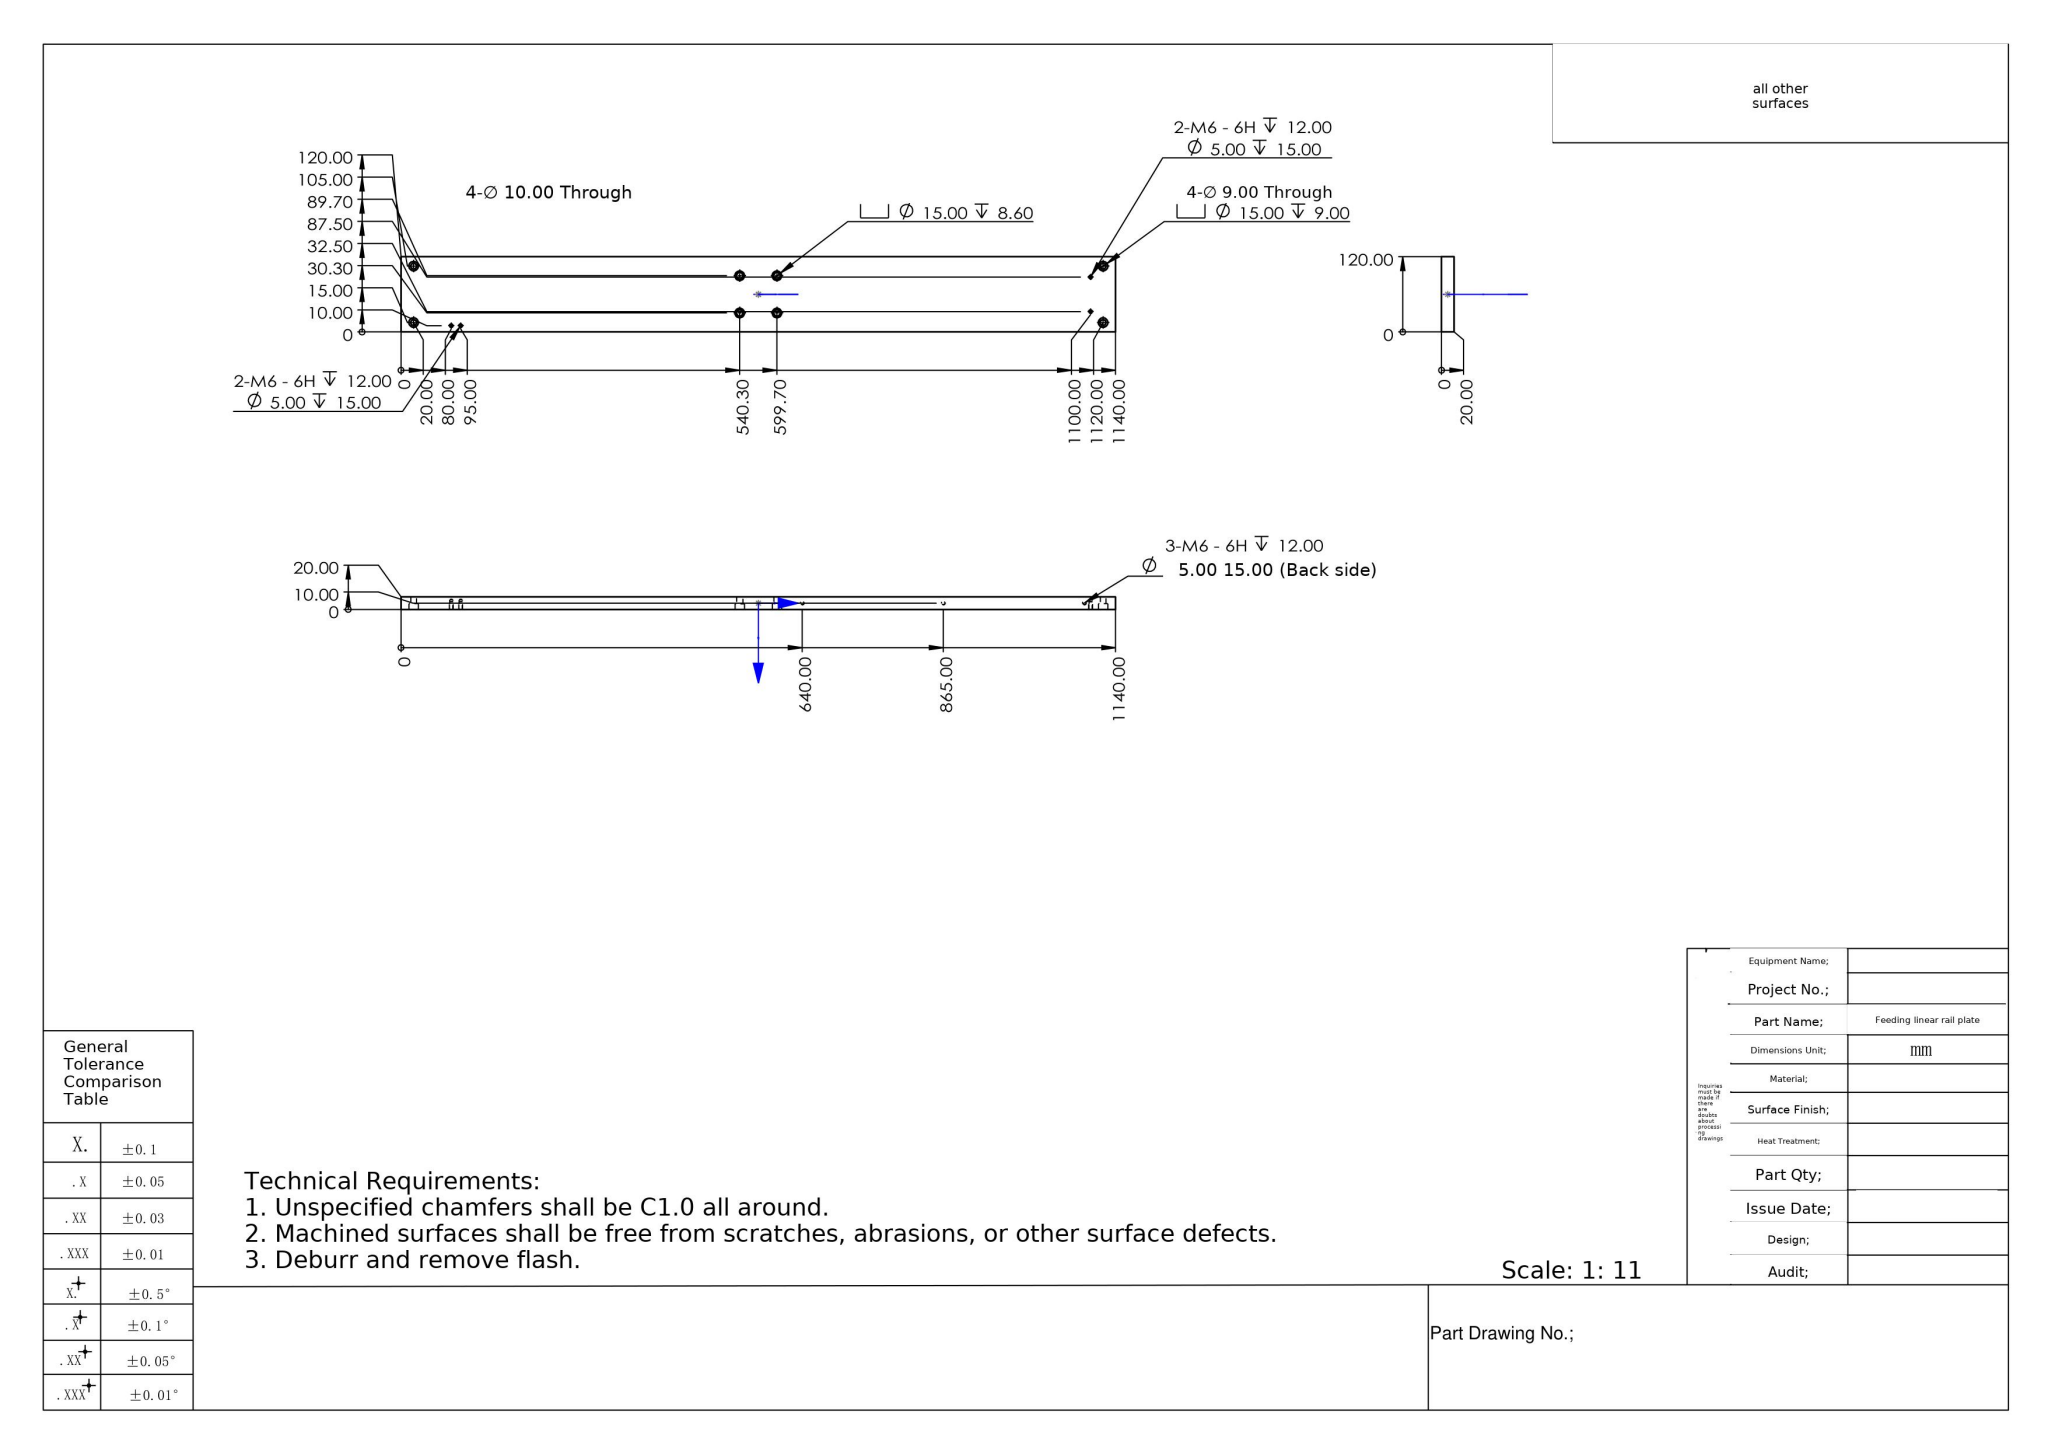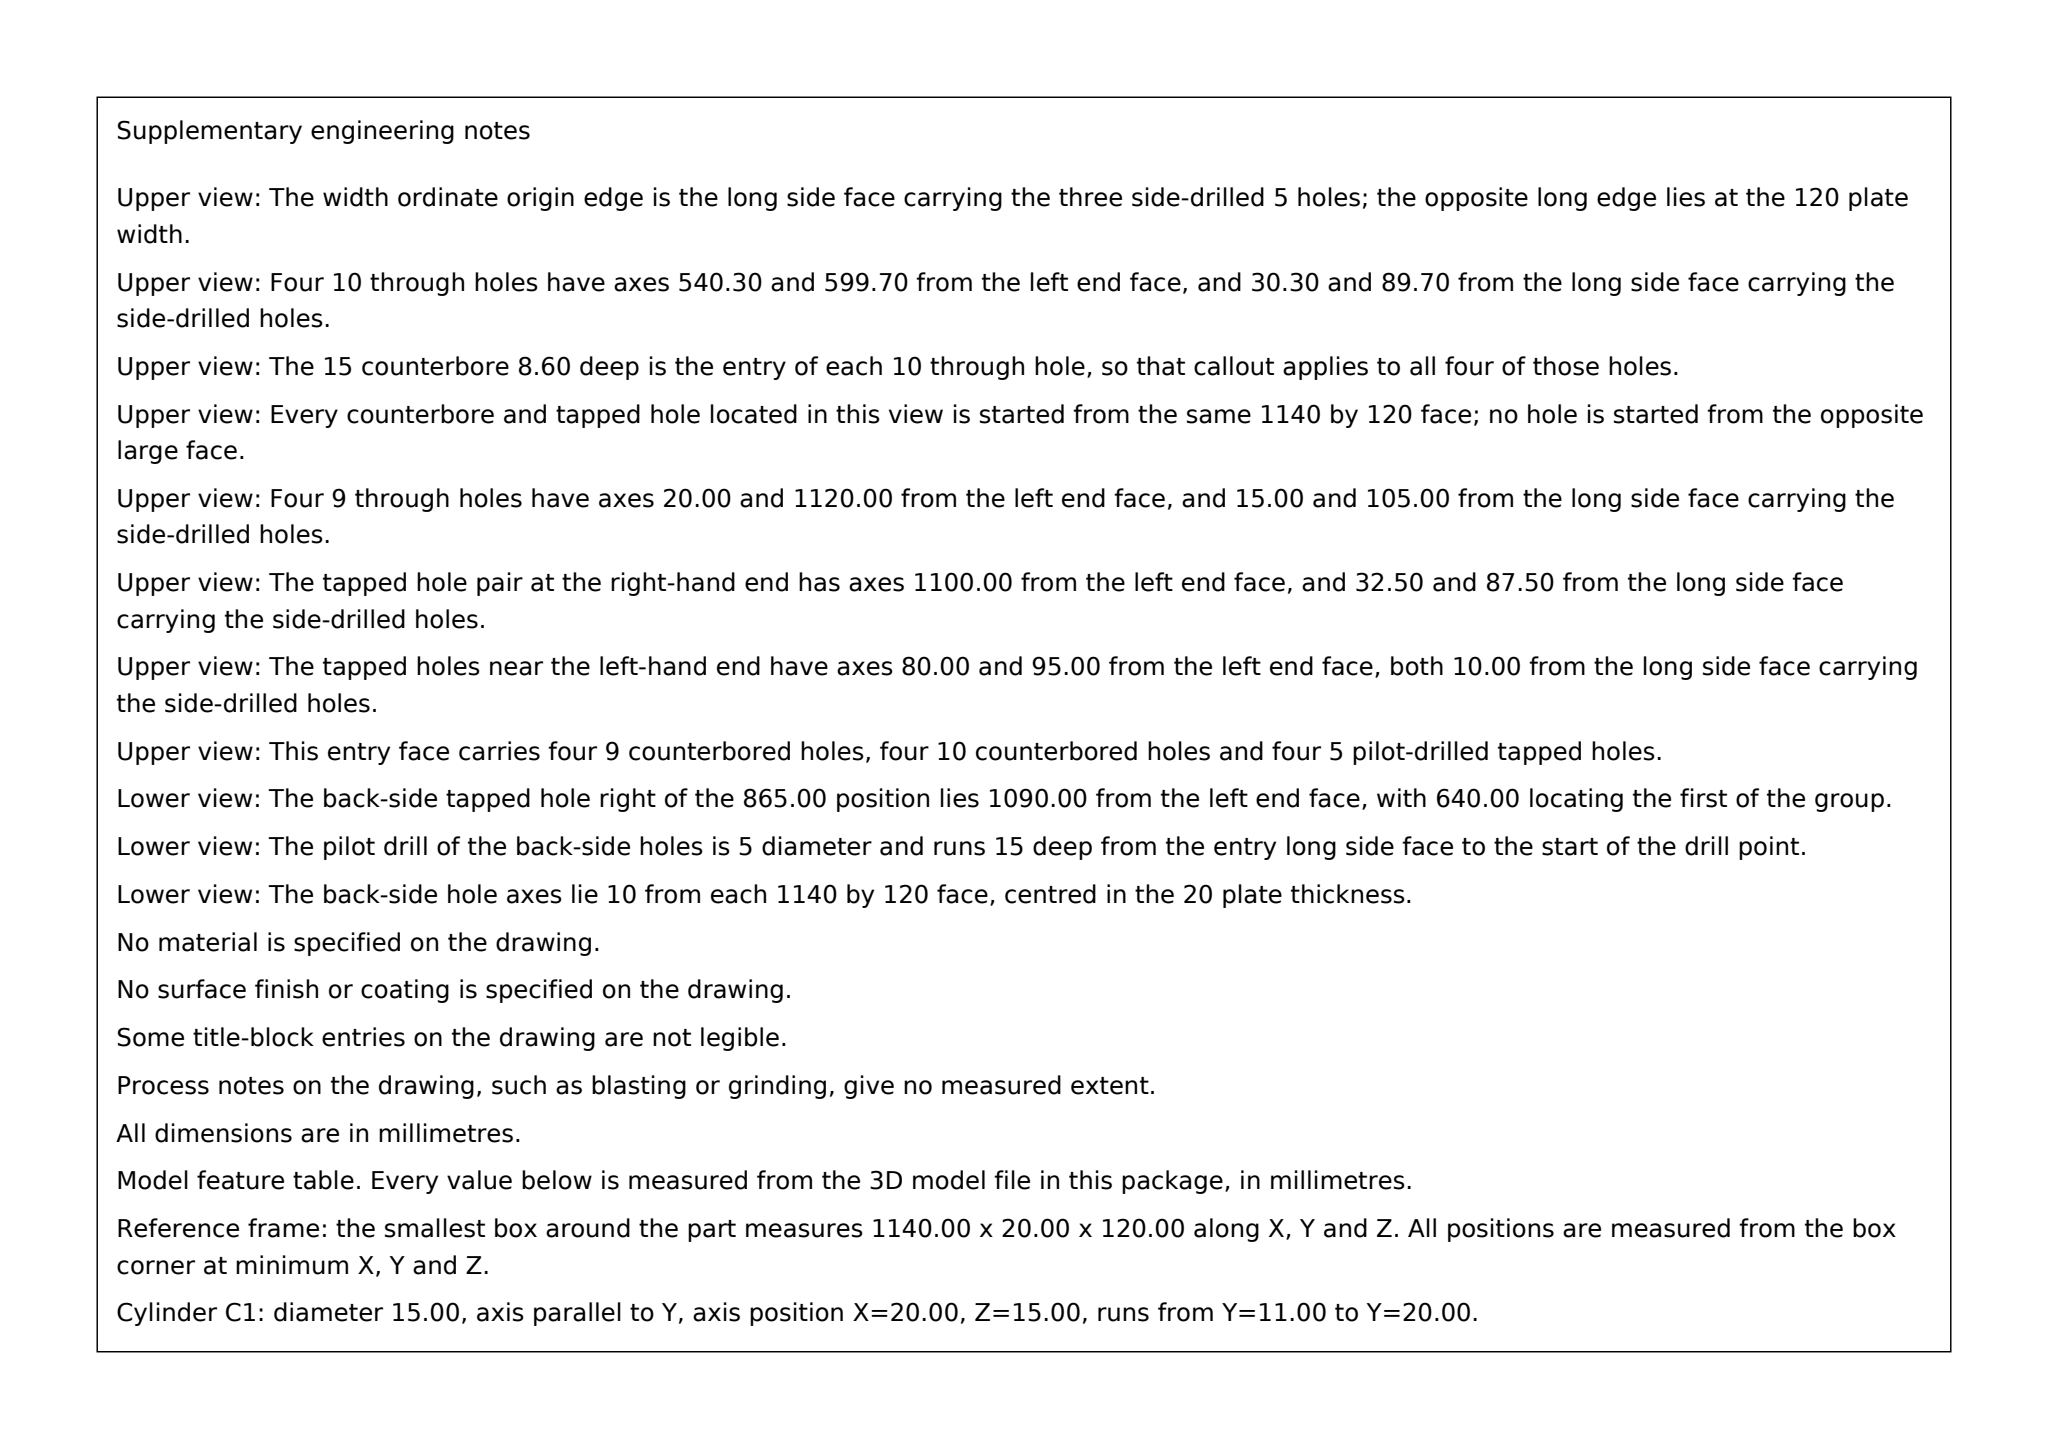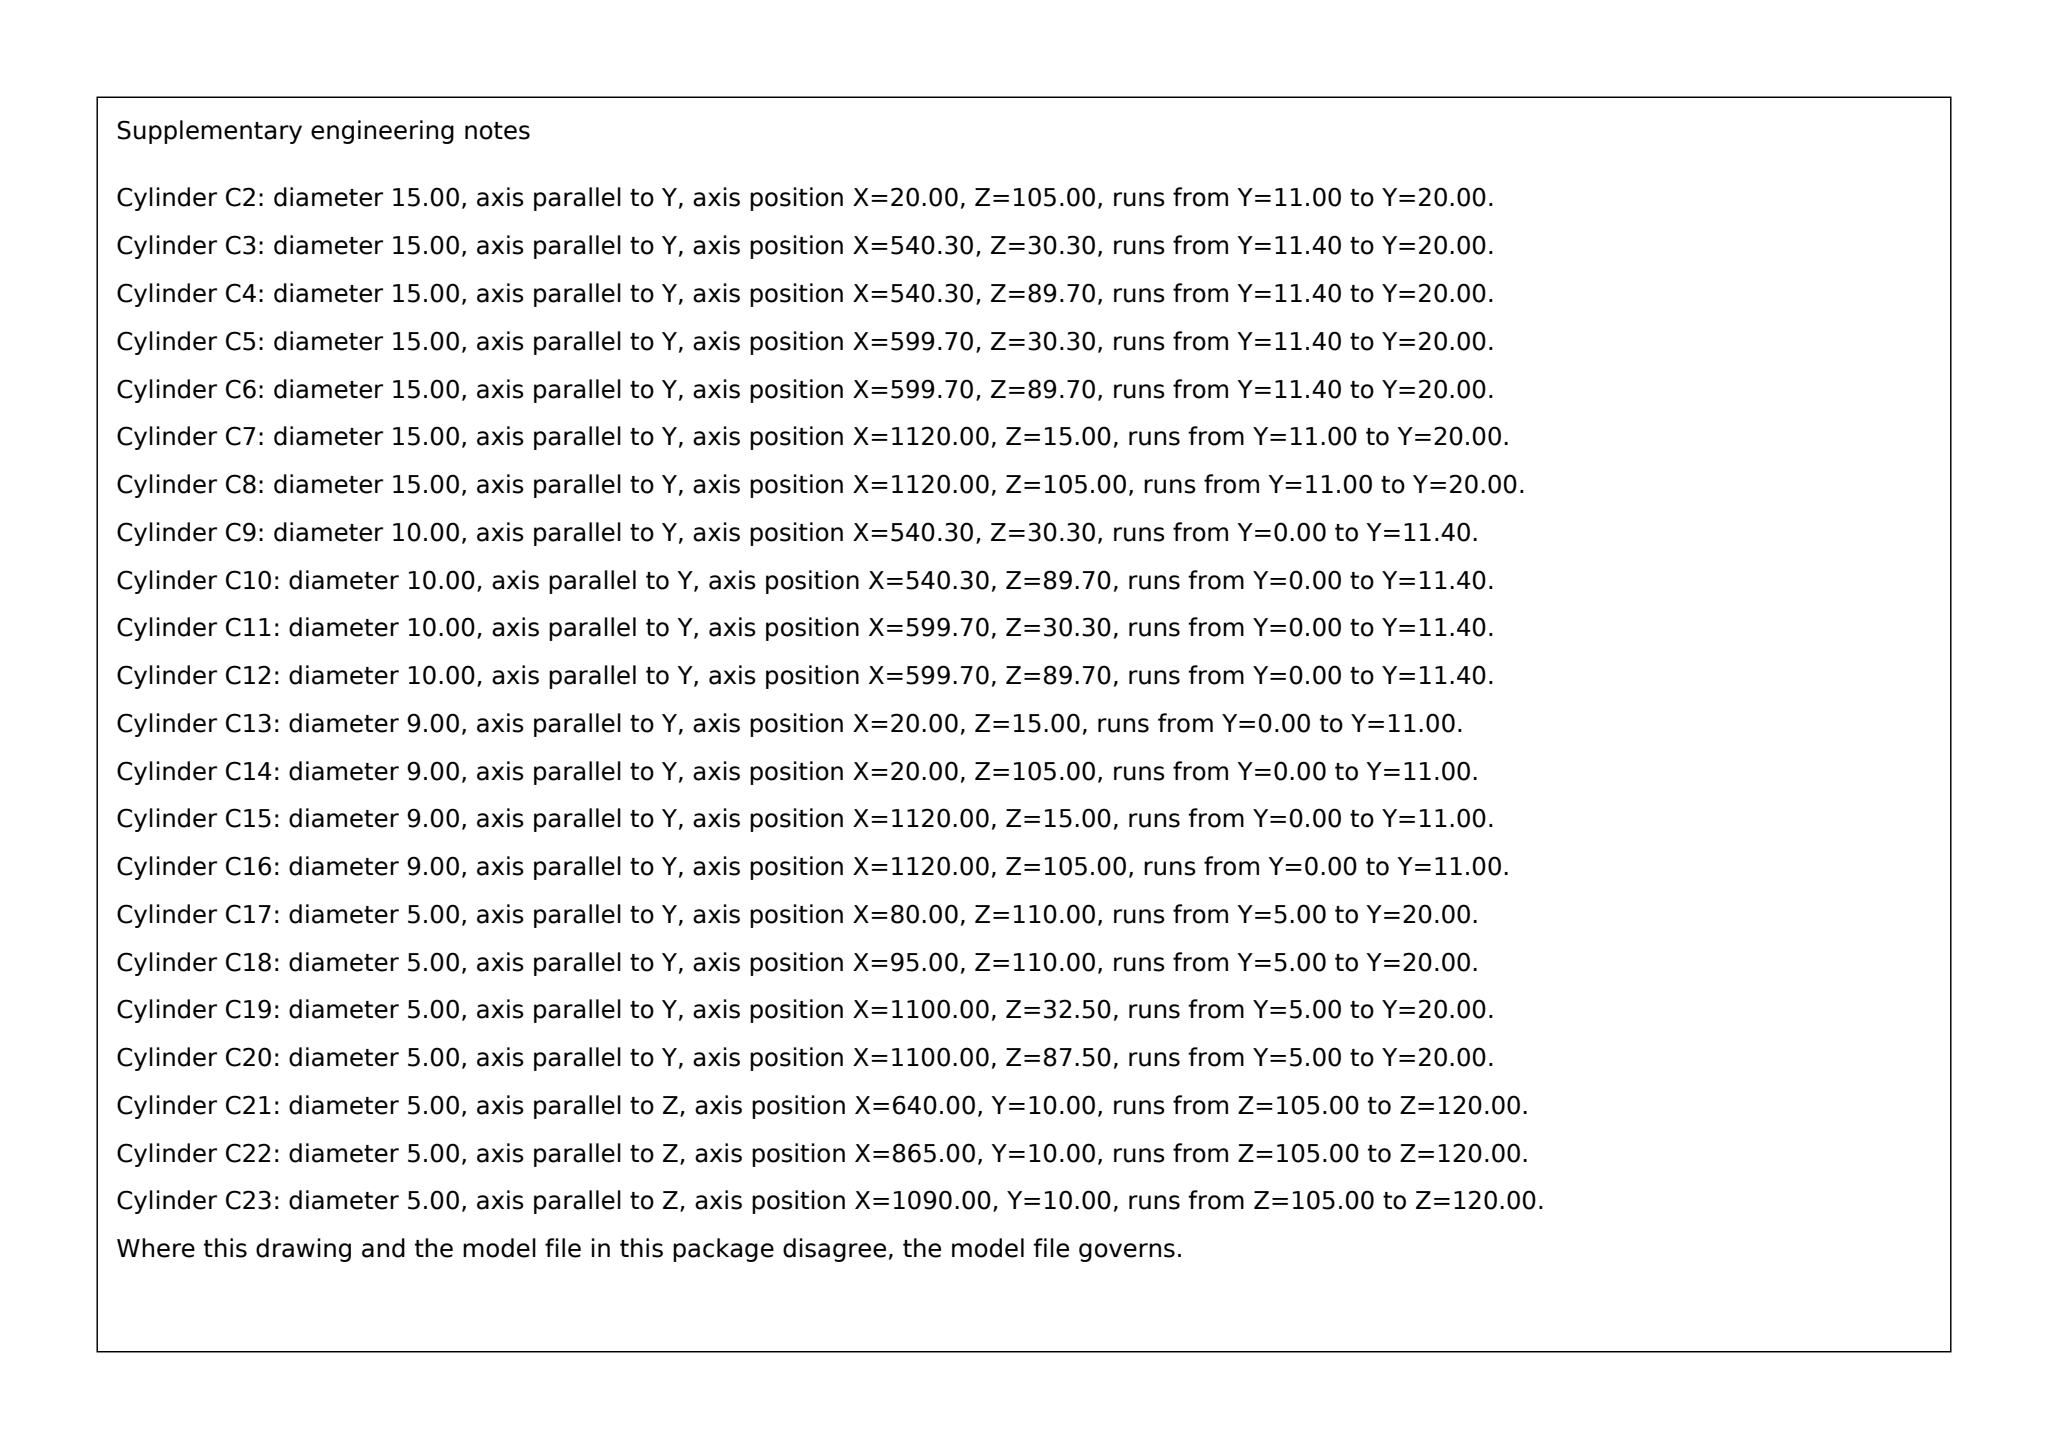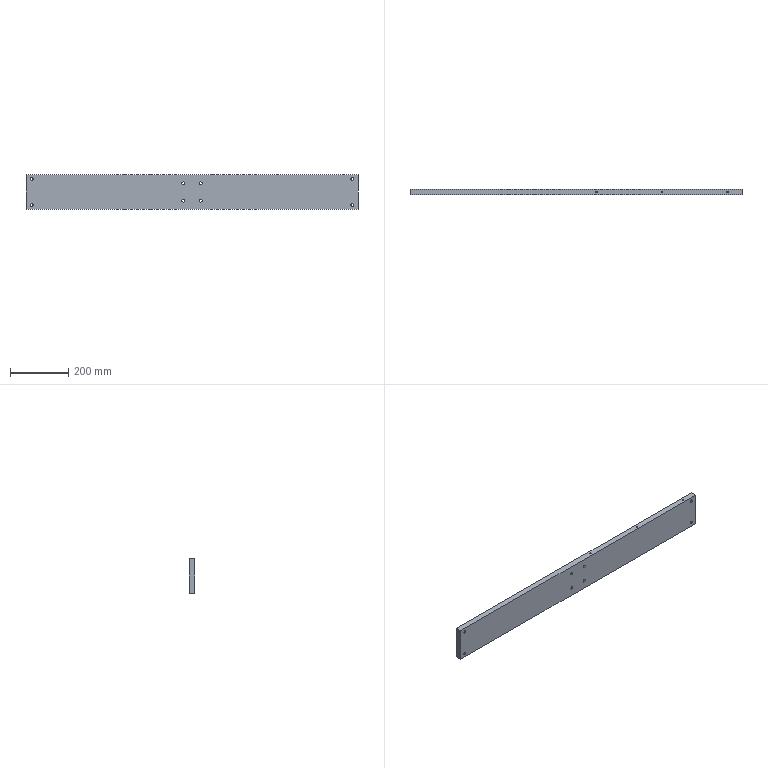Part | SolidWorks | mm | 1 solid | 74 faces | box 1140 x 20 x 120 mm | volume 2715048 mm3 | cylinder 46 | cone 14 | plane 14 | commonest cylinder face diameters 15 x16 5 x14 10 x8 9 x8
Drawing notes:
4X Ø9 C'BORE Ø15 DP 9.00 (AT X=20 & X=1120, Z=15 & Z=105) IS MACHINED FROM THE Y=20.00 FACE (C'BORE FLAT AT Y=11.00 FROM Y=0 DATUM FACE). | from the solid: cylinders [15.0,'y',[20.0,null,15.0],9.0] and [15.0,'y',[1120.0,null,105.0],9.0] with axis_planes ['y',11.0,4] = 20.00-9.00, so c'bores open at Y=20
3X M6-6H DP 12 / DRILL Ø5.00 DP 15.00, AXIS PARALLEL TO Z, AT X=640.00, 865.00, 1090.00, Y=10.00 FROM MIN CORNER. | from the solid: cylinders [5.0,'z',[640.0,10.0,null],15.0], [5.0,'z',[865.0,10.0,null],15.0], [5.0,'z',[1090.0,10.0,null],15.0]
4X M6-6H TAPPED HOLE DP 12 / DRILL Ø5.00 DP 15.00, AXIS PARALLEL TO Y, ENTERED FROM THE Y=20.00 FACE (DRILL BOTTOMS AT Y=5.00), AT X=80.00 & X=95.00 (Z=110.00) AND X=1100.00 (Z=32.50 & Z=87.50), ALL FROM MIN CORNER OF 1140 x 20 x 120 BODY | from the solid: cylinders: 4X dia 5.0 axis y at (80,-,110),(95,-,110),(1100,-,32.5),(1100,-,87.5) from y=5.0 to y=20.0; axis_planes y=20.0 full face
4X Ø10 THRU; CBORE Ø15 DP 8.6 FR Y=20 FACE (BACK SIDE) | from the solid: Ø10 y-holes y0→11.4 at X540.3/599.7, Z30.3/89.7; Ø15 y-bores y11.4→20 same axes (8.6 deep)
4X M6-6H DP 12; DRILL Ø5 DP 15; AXIS PARALLEL Y; FR Y=20 FACE | from the solid: Ø5 y-holes y5→20 (15 deep) at (1100,32.5),(1100,87.5),(80,110),(95,110)
M6 PARALLEL Y LOC: X80 & X95 @ Z110; X1100 @ Z32.5 & Z87.5 | from the solid: Ø5 y-axis hole positions [80,110],[95,110],[1100,32.5],[1100,87.5]
M6-6H DP 12; DRILL Ø5 DP 15; AXIS PARALLEL Z; X=1090, Y=10; FR Z=120 | from the solid: Ø5 z-hole at (1090,10), z105→120, 15 deep from Z=120 face
X=1090: 1 M6 HOLE ONLY - DELETE DUPLICATE CALLOUT | from the solid: only one Ø5 z-cylinder at (1090,10,z105-120) in model
3X M6-6H DP 12; Ø5 DP 15 (BACK) AT X=640, 865, 1090; Y=10 | from the solid: Ø5 z-holes at (640,10),(865,10),(1090,10), z105→120
X=1090 M6 AXIS PARALLEL Z, ENTERS Z=120 FACE, Y=10, 1 PLC | from the solid: z-axis Ø5 hole (1090,10) runs z105→120; entry at Z=120 plane
Ø5 DP 15 (BACK) APPLIES TO ALL 3 PARALLEL Z M6: X640/865/1090 | from the solid: three Ø5 z-holes each 15 deep from Z=120 face, Y=10
build123d program:
from build123d import *

# Parameters (mm, degrees)
SKETCH1_W                                            = 1140
SKETCH1_H                                            = 20
BOSS_EXTRUDE1_DEPTH                                  = 60
HOLE_SIZE_ACCORDING_TO_THE_TYPE_OF_HEX_S_D           = 9
HOLE_SIZE_ACCORDING_TO_THE_TYPE_OF_HEX_S_CBORE_D     = 15
HOLE_SIZE_ACCORDING_TO_THE_TYPE_OF_HEX_S_CBORE_DEPTH = 9
M6_TAPPED_HOLE1_D                                    = 5
M6_TAPPED_HOLE1_DEPTH                                = 15
M6_TAPPED_HOLE1_TIP                                  = 1.502
M8_HEX_SOCKET_HEAD_CAP_SCREW_CBORE1_D                = 10
M8_HEX_SOCKET_HEAD_CAP_SCREW_CBORE1_CBORE_D          = 15
M8_HEX_SOCKET_HEAD_CAP_SCREW_CBORE1_CBORE_DEPTH      = 8.6
M6_TAPPED_HOLE2_D                                    = 5
M6_TAPPED_HOLE2_DEPTH                                = 15
M6_TAPPED_HOLE2_TIP                                  = 1.502
M6_TAPPED_HOLE3_D                                    = 5
M6_TAPPED_HOLE3_DEPTH                                = 15
M6_TAPPED_HOLE3_TIP                                  = 1.502


with BuildPart() as part:
    # Sketch1 → Boss-Extrude1 (new, symmetric)
    with BuildSketch(Plane.XY):
        Rectangle(SKETCH1_W, SKETCH1_H)
    extrude(amount=BOSS_EXTRUDE1_DEPTH, both=True)

    # Hole Size according to the type of Hex S (through all)
    with Locations(Plane(origin=(0, 10, 0), x_dir=(1, 0, 0), z_dir=(0, 1, 0))):
        with Locations((-550, 45), (-550, -45), (550, 45), (550, -45)):
            CounterBoreHole(HOLE_SIZE_ACCORDING_TO_THE_TYPE_OF_HEX_S_D / 2, HOLE_SIZE_ACCORDING_TO_THE_TYPE_OF_HEX_S_CBORE_D / 2, HOLE_SIZE_ACCORDING_TO_THE_TYPE_OF_HEX_S_CBORE_DEPTH)

    # M6 Tapped Hole1
    with Locations(Plane.XY.offset(60)):
        with Locations((70, 0), (295, 0), (520, 0)):
            Hole(M6_TAPPED_HOLE1_D / 2, depth=M6_TAPPED_HOLE1_DEPTH)
            with Locations((0, 0, -(M6_TAPPED_HOLE1_DEPTH + M6_TAPPED_HOLE1_TIP / 2))):  # 118° drill point
                Cone(0, M6_TAPPED_HOLE1_D / 2, M6_TAPPED_HOLE1_TIP, mode=Mode.SUBTRACT)

    # M8 Hex Socket Head Cap Screw CBORE1 (through all)
    with Locations(Plane(origin=(0, 10, 0), x_dir=(1, 0, 0), z_dir=(0, 1, 0))):
        with Locations((29.698, 29.698), (29.698, -29.698), (-29.698, -29.698), (-29.698, 29.698)):
            CounterBoreHole(M8_HEX_SOCKET_HEAD_CAP_SCREW_CBORE1_D / 2, M8_HEX_SOCKET_HEAD_CAP_SCREW_CBORE1_CBORE_D / 2, M8_HEX_SOCKET_HEAD_CAP_SCREW_CBORE1_CBORE_DEPTH)

    # M6 Tapped Hole2
    with Locations(Plane(origin=(23.67, 10, 26.577), x_dir=(1, 0, 0), z_dir=(0, 1, 0))):
        with Locations((-513.67, -23.423), (-498.67, -23.423)):
            Hole(M6_TAPPED_HOLE2_D / 2, depth=M6_TAPPED_HOLE2_DEPTH)
            with Locations((0, 0, -(M6_TAPPED_HOLE2_DEPTH + M6_TAPPED_HOLE2_TIP / 2))):  # 118° drill point
                Cone(0, M6_TAPPED_HOLE2_D / 2, M6_TAPPED_HOLE2_TIP, mode=Mode.SUBTRACT)

    # M6 Tapped Hole3
    with Locations(Plane(origin=(0, 10, 0), x_dir=(1, 0, 0), z_dir=(0, 1, 0))):
        with Locations((530, 27.5), (530, -27.5)):
            Hole(M6_TAPPED_HOLE3_D / 2, depth=M6_TAPPED_HOLE3_DEPTH)
            with Locations((0, 0, -(M6_TAPPED_HOLE3_DEPTH + M6_TAPPED_HOLE3_TIP / 2))):  # 118° drill point
                Cone(0, M6_TAPPED_HOLE3_D / 2, M6_TAPPED_HOLE3_TIP, mode=Mode.SUBTRACT)


solid = part.part